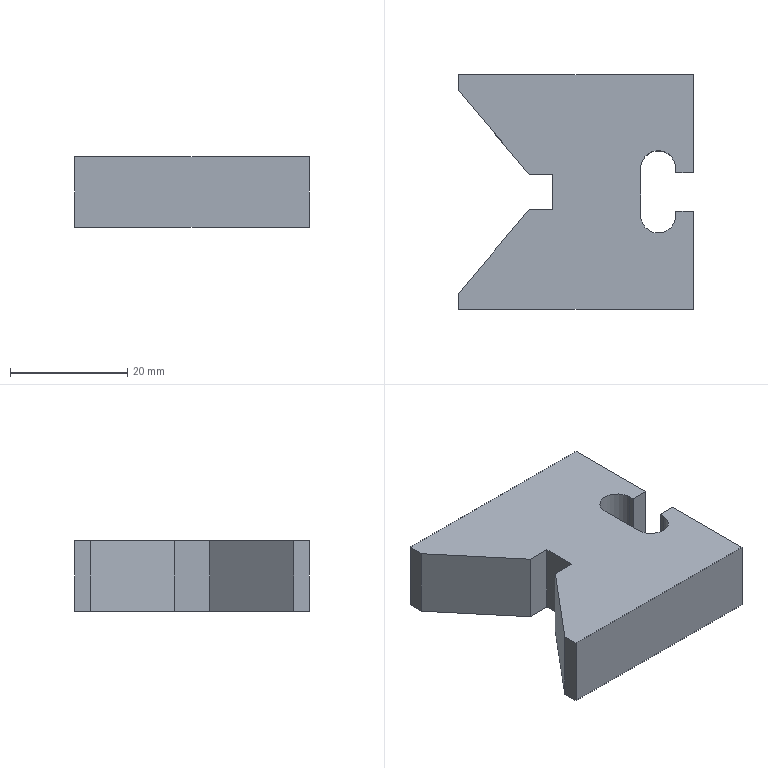Component | NX | MOV_V_BLOCK | 1 solid | 20 faces | volume 14840 mm3 | plane 18 | cylinder 2 | commonest cylinder face diameters 6 x2